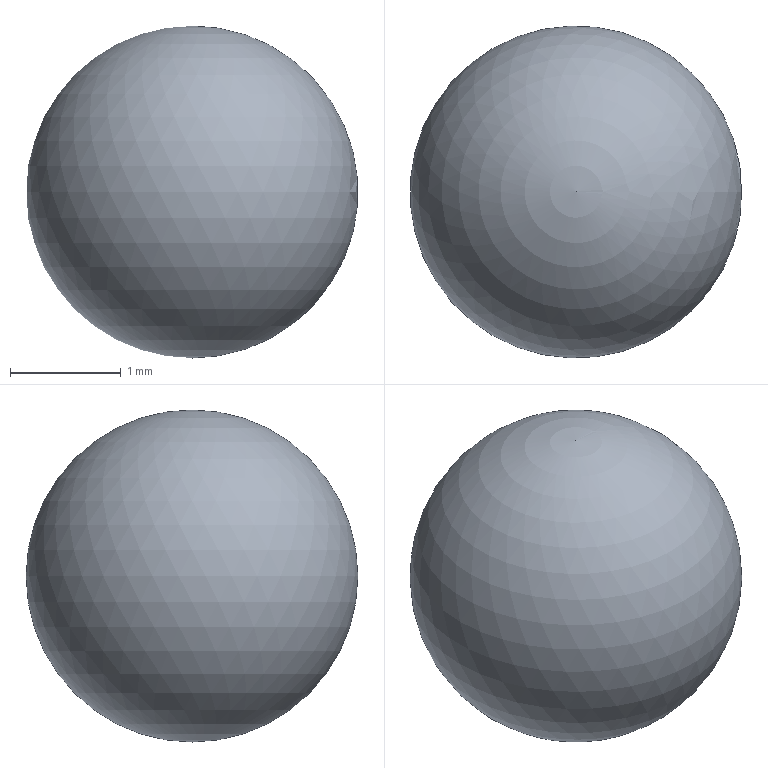Component | NX | 13_STEEL_BALL_2 | 1 solid | 1 faces | box 3 x 3 x 3 mm | volume 14 mm3 | sphere 1
STEP:
#1=CARTESIAN_POINT('',(0.,0.,0.));
#2=DIRECTION('',(0.,0.,1.));
#3=DIRECTION('',(1.,0.,0.));
#4=AXIS2_PLACEMENT_3D('',#1,#2,#3);
#5=CARTESIAN_POINT('',(-59.084,201.112,-226.719));
#6=VERTEX_POINT('',#5);
#7=VERTEX_LOOP('',#6);
#8=FACE_BOUND('',#7,.T.);
#9=CARTESIAN_POINT('',(-59.084,201.112,-225.219));
#10=DIRECTION('',(0.,0.,1.));
#11=DIRECTION('',(1.,0.,0.));
#12=AXIS2_PLACEMENT_3D('',#9,#10,#11);
#13=SPHERICAL_SURFACE('',#12,1.5);
#14=ADVANCED_FACE('',(#8),#13,.T.);
#15=CLOSED_SHELL('',(#14));
#16=MANIFOLD_SOLID_BREP('',#15);
#17=(LENGTH_UNIT()NAMED_UNIT(*)SI_UNIT(.MILLI.,.METRE.));
#18=UNCERTAINTY_MEASURE_WITH_UNIT(LENGTH_MEASURE(0.0000001),#17,'','');
#19=(NAMED_UNIT(*)PLANE_ANGLE_UNIT()SI_UNIT($,.RADIAN.));
#20=(NAMED_UNIT(*)SI_UNIT($,.STERADIAN.)SOLID_ANGLE_UNIT());
#21=(GEOMETRIC_REPRESENTATION_CONTEXT(3)GLOBAL_UNCERTAINTY_ASSIGNED_CONTEXT((#18))GLOBAL_UNIT_ASSIGNED_CONTEXT((#17,#19,#20))REPRESENTATION_CONTEXT('',''));
#22=ADVANCED_BREP_SHAPE_REPRESENTATION('',(#4,#16),#21);